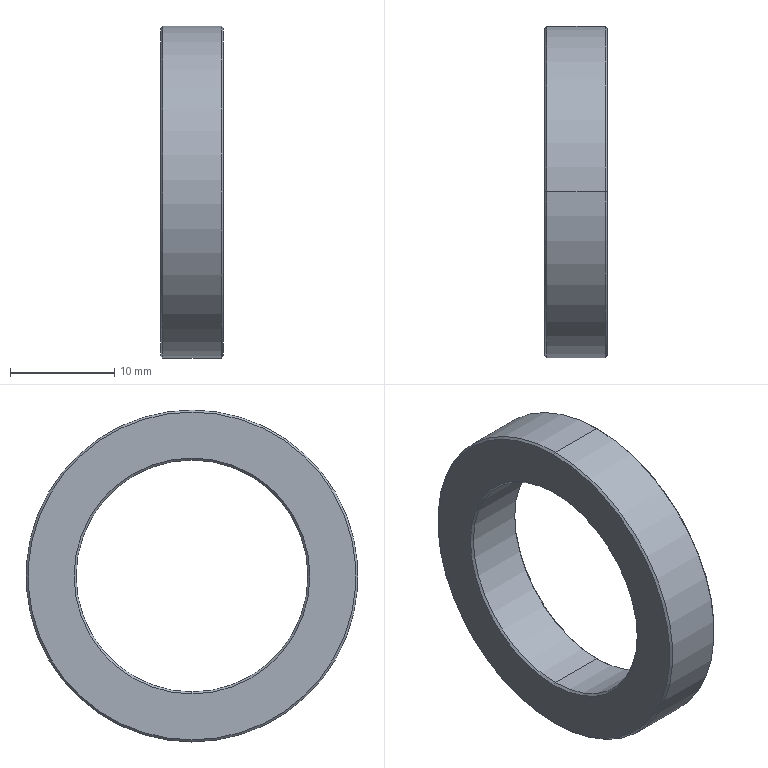Component | SolidWorks | XXXXX08-01-040514RotaryDriveShaft-1_XXXXX08-01-040515-1 | 1 solid | 14 faces | box 6 x 31.8 x 31.8 mm | volume 2436 mm3 | cone 8 | cylinder 4 | plane 2 | commonest cylinder face diameters 22.2 x2 31.8 x2 | material 45
build123d program:
from build123d import *

# Parameters (mm, degrees)
SKETCH1_R           = 15.9
SKETCH1_R_2         = 11.1
BOSS_EXTRUDE1_DEPTH = 3
CHAMFER1_SIZE       = 0.2


with BuildPart() as part:
    # Sketch1 → Boss-Extrude1 (new, symmetric)
    with BuildSketch(Plane(origin=(0, 0, 0), x_dir=(0, 0, -1), z_dir=(1, 0, 0))):
        Circle(SKETCH1_R)
        Circle(SKETCH1_R_2, mode=Mode.SUBTRACT)
    extrude(amount=BOSS_EXTRUDE1_DEPTH, both=True)

    # Chamfer1
    chamfer1_edges = [part.edges().sort_by_distance(p)[0] for p in [
        (-3, 0, 15.9),
        (3, 0, 15.9),
        (-3, 0, 11.1),
        (3, 0, 11.1),
    ]]
    chamfer(chamfer1_edges, length=CHAMFER1_SIZE)


solid = part.part

# Placed as in the assembly
solid = solid.moved(Location((-32.7, 0, 0), (0, 0, 0)))
STEP:
#1=COLOUR_RGB('',0.7922,0.8196,0.9333);
#2=FILL_AREA_STYLE_COLOUR('',#1);
#3=FILL_AREA_STYLE('',(#2));
#4=SURFACE_STYLE_FILL_AREA(#3);
#5=SURFACE_SIDE_STYLE('',(#4));
#6=SURFACE_STYLE_USAGE(.BOTH.,#5);
#7=PRESENTATION_STYLE_ASSIGNMENT((#6));
#8=CARTESIAN_POINT('',(-1.177,0.,0.437));
#9=VERTEX_POINT('',#8);
#10=CARTESIAN_POINT('',(-1.177,0.,-0.437));
#11=VERTEX_POINT('',#10);
#12=CARTESIAN_POINT('',(-1.177,0.,-0.));
#13=DIRECTION('',(1.,0.,0.));
#14=DIRECTION('',(0.,0.,-1.));
#15=AXIS2_PLACEMENT_3D('',#12,#13,#14);
#16=CIRCLE('',#15,0.437);
#17=EDGE_CURVE('',#9,#11,#16,.T.);
#18=ORIENTED_EDGE('',*,*,#17,.F.);
#19=CARTESIAN_POINT('',(-1.169,0.,0.4449));
#20=VERTEX_POINT('',#19);
#21=CARTESIAN_POINT('',(-1.177,0.,0.437));
#22=DIRECTION('',(0.7071,0.,0.7071));
#23=VECTOR('',#22,39.37);
#24=LINE('',#21,#23);
#25=EDGE_CURVE('',#9,#20,#24,.T.);
#26=ORIENTED_EDGE('',*,*,#25,.T.);
#27=CARTESIAN_POINT('',(-1.169,0.,-0.4449));
#28=VERTEX_POINT('',#27);
#29=CARTESIAN_POINT('',(-1.169,0.,-0.));
#30=DIRECTION('',(-1.,0.,0.));
#31=DIRECTION('',(0.,0.,-1.));
#32=AXIS2_PLACEMENT_3D('',#29,#30,#31);
#33=CIRCLE('',#32,0.4449);
#34=EDGE_CURVE('',#28,#20,#33,.T.);
#35=ORIENTED_EDGE('',*,*,#34,.F.);
#36=CARTESIAN_POINT('',(-1.177,0.,-0.437));
#37=DIRECTION('',(0.7071,0.,-0.7071));
#38=VECTOR('',#37,39.37);
#39=LINE('',#36,#38);
#40=EDGE_CURVE('',#11,#28,#39,.T.);
#41=ORIENTED_EDGE('',*,*,#40,.F.);
#42=EDGE_LOOP('',(#18,#26,#35,#41));
#43=FACE_OUTER_BOUND('',#42,.T.);
#44=CARTESIAN_POINT('',(-1.177,0.,-0.));
#45=DIRECTION('',(1.,0.,0.));
#46=DIRECTION('',(0.,0.,-1.));
#47=AXIS2_PLACEMENT_3D('',#44,#45,#46);
#48=CONICAL_SURFACE('',#47,0.437,0.7854);
#49=ADVANCED_FACE('',(#43),#48,.F.);
#50=CARTESIAN_POINT('',(-1.398,0.,-0.437));
#51=VERTEX_POINT('',#50);
#52=CARTESIAN_POINT('',(-1.398,0.,0.437));
#53=VERTEX_POINT('',#52);
#54=CARTESIAN_POINT('',(-1.398,0.,-0.));
#55=DIRECTION('',(-1.,0.,0.));
#56=DIRECTION('',(0.,0.,-1.));
#57=AXIS2_PLACEMENT_3D('',#54,#55,#56);
#58=CIRCLE('',#57,0.437);
#59=EDGE_CURVE('',#51,#53,#58,.T.);
#60=ORIENTED_EDGE('',*,*,#59,.F.);
#61=CARTESIAN_POINT('',(-1.406,0.,-0.4449));
#62=VERTEX_POINT('',#61);
#63=CARTESIAN_POINT('',(-1.406,0.,-0.4449));
#64=DIRECTION('',(-0.7071,0.,-0.7071));
#65=VECTOR('',#64,39.37);
#66=LINE('',#63,#65);
#67=EDGE_CURVE('',#51,#62,#66,.T.);
#68=ORIENTED_EDGE('',*,*,#67,.T.);
#69=CARTESIAN_POINT('',(-1.406,0.,0.4449));
#70=VERTEX_POINT('',#69);
#71=CARTESIAN_POINT('',(-1.406,0.,-0.));
#72=DIRECTION('',(1.,0.,0.));
#73=DIRECTION('',(0.,0.,-1.));
#74=AXIS2_PLACEMENT_3D('',#71,#72,#73);
#75=CIRCLE('',#74,0.4449);
#76=EDGE_CURVE('',#70,#62,#75,.T.);
#77=ORIENTED_EDGE('',*,*,#76,.F.);
#78=CARTESIAN_POINT('',(-1.406,0.,0.4449));
#79=DIRECTION('',(-0.7071,0.,0.7071));
#80=VECTOR('',#79,39.37);
#81=LINE('',#78,#80);
#82=EDGE_CURVE('',#53,#70,#81,.T.);
#83=ORIENTED_EDGE('',*,*,#82,.F.);
#84=EDGE_LOOP('',(#60,#68,#77,#83));
#85=FACE_OUTER_BOUND('',#84,.T.);
#86=CARTESIAN_POINT('',(-1.406,0.,-0.));
#87=DIRECTION('',(-1.,0.,0.));
#88=DIRECTION('',(0.,0.,1.));
#89=AXIS2_PLACEMENT_3D('',#86,#87,#88);
#90=CONICAL_SURFACE('',#89,0.4449,0.7854);
#91=ADVANCED_FACE('',(#85),#90,.F.);
#92=CARTESIAN_POINT('',(-1.169,0.,-0.6181));
#93=VERTEX_POINT('',#92);
#94=CARTESIAN_POINT('',(-1.169,0.,0.6181));
#95=VERTEX_POINT('',#94);
#96=CARTESIAN_POINT('',(-1.169,0.,-0.));
#97=DIRECTION('',(1.,0.,0.));
#98=DIRECTION('',(0.,0.,-1.));
#99=AXIS2_PLACEMENT_3D('',#96,#97,#98);
#100=CIRCLE('',#99,0.6181);
#101=EDGE_CURVE('',#93,#95,#100,.T.);
#102=ORIENTED_EDGE('',*,*,#101,.F.);
#103=CARTESIAN_POINT('',(-1.177,0.,-0.626));
#104=VERTEX_POINT('',#103);
#105=CARTESIAN_POINT('',(-1.169,0.,-0.6181));
#106=DIRECTION('',(-0.7071,0.,-0.7071));
#107=VECTOR('',#106,39.37);
#108=LINE('',#105,#107);
#109=EDGE_CURVE('',#93,#104,#108,.T.);
#110=ORIENTED_EDGE('',*,*,#109,.T.);
#111=CARTESIAN_POINT('',(-1.177,0.,0.626));
#112=VERTEX_POINT('',#111);
#113=CARTESIAN_POINT('',(-1.177,0.,-0.));
#114=DIRECTION('',(-1.,0.,0.));
#115=DIRECTION('',(0.,0.,-1.));
#116=AXIS2_PLACEMENT_3D('',#113,#114,#115);
#117=CIRCLE('',#116,0.626);
#118=EDGE_CURVE('',#112,#104,#117,.T.);
#119=ORIENTED_EDGE('',*,*,#118,.F.);
#120=CARTESIAN_POINT('',(-1.169,0.,0.6181));
#121=DIRECTION('',(-0.7071,0.,0.7071));
#122=VECTOR('',#121,39.37);
#123=LINE('',#120,#122);
#124=EDGE_CURVE('',#95,#112,#123,.T.);
#125=ORIENTED_EDGE('',*,*,#124,.F.);
#126=EDGE_LOOP('',(#102,#110,#119,#125));
#127=FACE_OUTER_BOUND('',#126,.T.);
#128=CARTESIAN_POINT('',(-1.169,0.,-0.));
#129=DIRECTION('',(-1.,0.,0.));
#130=DIRECTION('',(0.,0.,1.));
#131=AXIS2_PLACEMENT_3D('',#128,#129,#130);
#132=CONICAL_SURFACE('',#131,0.6181,0.7854);
#133=ADVANCED_FACE('',(#127),#132,.T.);
#134=CARTESIAN_POINT('',(-1.406,0.,0.6181));
#135=VERTEX_POINT('',#134);
#136=CARTESIAN_POINT('',(-1.406,0.,-0.6181));
#137=VERTEX_POINT('',#136);
#138=CARTESIAN_POINT('',(-1.406,0.,-0.));
#139=DIRECTION('',(-1.,0.,0.));
#140=DIRECTION('',(0.,0.,-1.));
#141=AXIS2_PLACEMENT_3D('',#138,#139,#140);
#142=CIRCLE('',#141,0.6181);
#143=EDGE_CURVE('',#135,#137,#142,.T.);
#144=ORIENTED_EDGE('',*,*,#143,.F.);
#145=CARTESIAN_POINT('',(-1.398,0.,0.626));
#146=VERTEX_POINT('',#145);
#147=CARTESIAN_POINT('',(-1.398,0.,0.626));
#148=DIRECTION('',(0.7071,0.,0.7071));
#149=VECTOR('',#148,39.37);
#150=LINE('',#147,#149);
#151=EDGE_CURVE('',#135,#146,#150,.T.);
#152=ORIENTED_EDGE('',*,*,#151,.T.);
#153=CARTESIAN_POINT('',(-1.398,0.,-0.626));
#154=VERTEX_POINT('',#153);
#155=CARTESIAN_POINT('',(-1.398,0.,-0.));
#156=DIRECTION('',(1.,0.,0.));
#157=DIRECTION('',(0.,0.,-1.));
#158=AXIS2_PLACEMENT_3D('',#155,#156,#157);
#159=CIRCLE('',#158,0.626);
#160=EDGE_CURVE('',#154,#146,#159,.T.);
#161=ORIENTED_EDGE('',*,*,#160,.F.);
#162=CARTESIAN_POINT('',(-1.398,0.,-0.626));
#163=DIRECTION('',(0.7071,0.,-0.7071));
#164=VECTOR('',#163,39.37);
#165=LINE('',#162,#164);
#166=EDGE_CURVE('',#137,#154,#165,.T.);
#167=ORIENTED_EDGE('',*,*,#166,.F.);
#168=EDGE_LOOP('',(#144,#152,#161,#167));
#169=FACE_OUTER_BOUND('',#168,.T.);
#170=CARTESIAN_POINT('',(-1.398,0.,-0.));
#171=DIRECTION('',(1.,0.,0.));
#172=DIRECTION('',(0.,0.,-1.));
#173=AXIS2_PLACEMENT_3D('',#170,#171,#172);
#174=CONICAL_SURFACE('',#173,0.626,0.7854);
#175=ADVANCED_FACE('',(#169),#174,.T.);
#176=ORIENTED_EDGE('',*,*,#17,.T.);
#177=CARTESIAN_POINT('',(-1.169,0.,-0.437));
#178=DIRECTION('',(-1.,0.,0.));
#179=VECTOR('',#178,39.37);
#180=LINE('',#177,#179);
#181=EDGE_CURVE('',#11,#51,#180,.T.);
#182=ORIENTED_EDGE('',*,*,#181,.T.);
#183=ORIENTED_EDGE('',*,*,#59,.T.);
#184=CARTESIAN_POINT('',(-1.169,0.,0.437));
#185=DIRECTION('',(-1.,0.,0.));
#186=VECTOR('',#185,39.37);
#187=LINE('',#184,#186);
#188=EDGE_CURVE('',#9,#53,#187,.T.);
#189=ORIENTED_EDGE('',*,*,#188,.F.);
#190=EDGE_LOOP('',(#176,#182,#183,#189));
#191=FACE_OUTER_BOUND('',#190,.T.);
#192=CARTESIAN_POINT('',(-1.169,0.,-0.));
#193=DIRECTION('',(-1.,0.,0.));
#194=DIRECTION('',(0.,0.,1.));
#195=AXIS2_PLACEMENT_3D('',#192,#193,#194);
#196=CYLINDRICAL_SURFACE('',#195,0.437);
#197=ADVANCED_FACE('',(#191),#196,.F.);
#198=ORIENTED_EDGE('',*,*,#118,.T.);
#199=CARTESIAN_POINT('',(-1.169,0.,-0.626));
#200=DIRECTION('',(-1.,0.,0.));
#201=VECTOR('',#200,39.37);
#202=LINE('',#199,#201);
#203=EDGE_CURVE('',#104,#154,#202,.T.);
#204=ORIENTED_EDGE('',*,*,#203,.T.);
#205=ORIENTED_EDGE('',*,*,#160,.T.);
#206=CARTESIAN_POINT('',(-1.169,0.,0.626));
#207=DIRECTION('',(-1.,0.,0.));
#208=VECTOR('',#207,39.37);
#209=LINE('',#206,#208);
#210=EDGE_CURVE('',#112,#146,#209,.T.);
#211=ORIENTED_EDGE('',*,*,#210,.F.);
#212=EDGE_LOOP('',(#198,#204,#205,#211));
#213=FACE_OUTER_BOUND('',#212,.T.);
#214=CARTESIAN_POINT('',(-1.169,0.,-0.));
#215=DIRECTION('',(-1.,0.,0.));
#216=DIRECTION('',(0.,0.,1.));
#217=AXIS2_PLACEMENT_3D('',#214,#215,#216);
#218=CYLINDRICAL_SURFACE('',#217,0.626);
#219=ADVANCED_FACE('',(#213),#218,.T.);
#220=CARTESIAN_POINT('',(-1.169,0.,-0.));
#221=DIRECTION('',(1.,0.,0.));
#222=DIRECTION('',(0.,0.,-1.));
#223=AXIS2_PLACEMENT_3D('',#220,#221,#222);
#224=CIRCLE('',#223,0.6181);
#225=EDGE_CURVE('',#95,#93,#224,.T.);
#226=ORIENTED_EDGE('',*,*,#225,.T.);
#227=ORIENTED_EDGE('',*,*,#101,.T.);
#228=EDGE_LOOP('',(#226,#227));
#229=FACE_OUTER_BOUND('',#228,.T.);
#230=ORIENTED_EDGE('',*,*,#34,.T.);
#231=CARTESIAN_POINT('',(-1.169,0.,-0.));
#232=DIRECTION('',(-1.,0.,0.));
#233=DIRECTION('',(0.,0.,-1.));
#234=AXIS2_PLACEMENT_3D('',#231,#232,#233);
#235=CIRCLE('',#234,0.4449);
#236=EDGE_CURVE('',#20,#28,#235,.T.);
#237=ORIENTED_EDGE('',*,*,#236,.T.);
#238=EDGE_LOOP('',(#230,#237));
#239=FACE_BOUND('',#238,.T.);
#240=CARTESIAN_POINT('',(-1.169,0.,-0.));
#241=DIRECTION('',(1.,0.,0.));
#242=DIRECTION('',(0.,0.,-1.));
#243=AXIS2_PLACEMENT_3D('',#240,#241,#242);
#244=PLANE('',#243);
#245=ADVANCED_FACE('',(#229,#239),#244,.T.);
#246=CARTESIAN_POINT('',(-1.406,0.,-0.));
#247=DIRECTION('',(-1.,0.,0.));
#248=DIRECTION('',(0.,0.,-1.));
#249=AXIS2_PLACEMENT_3D('',#246,#247,#248);
#250=CIRCLE('',#249,0.6181);
#251=EDGE_CURVE('',#137,#135,#250,.T.);
#252=ORIENTED_EDGE('',*,*,#251,.T.);
#253=ORIENTED_EDGE('',*,*,#143,.T.);
#254=EDGE_LOOP('',(#252,#253));
#255=FACE_OUTER_BOUND('',#254,.T.);
#256=ORIENTED_EDGE('',*,*,#76,.T.);
#257=CARTESIAN_POINT('',(-1.406,0.,-0.));
#258=DIRECTION('',(1.,0.,0.));
#259=DIRECTION('',(0.,0.,-1.));
#260=AXIS2_PLACEMENT_3D('',#257,#258,#259);
#261=CIRCLE('',#260,0.4449);
#262=EDGE_CURVE('',#62,#70,#261,.T.);
#263=ORIENTED_EDGE('',*,*,#262,.T.);
#264=EDGE_LOOP('',(#256,#263));
#265=FACE_BOUND('',#264,.T.);
#266=CARTESIAN_POINT('',(-1.406,0.,-0.));
#267=DIRECTION('',(1.,0.,0.));
#268=DIRECTION('',(0.,0.,-1.));
#269=AXIS2_PLACEMENT_3D('',#266,#267,#268);
#270=PLANE('',#269);
#271=ADVANCED_FACE('',(#255,#265),#270,.F.);
#272=ORIENTED_EDGE('',*,*,#203,.F.);
#273=CARTESIAN_POINT('',(-1.177,0.,-0.));
#274=DIRECTION('',(-1.,0.,0.));
#275=DIRECTION('',(0.,0.,-1.));
#276=AXIS2_PLACEMENT_3D('',#273,#274,#275);
#277=CIRCLE('',#276,0.626);
#278=EDGE_CURVE('',#104,#112,#277,.T.);
#279=ORIENTED_EDGE('',*,*,#278,.T.);
#280=ORIENTED_EDGE('',*,*,#210,.T.);
#281=CARTESIAN_POINT('',(-1.398,0.,-0.));
#282=DIRECTION('',(1.,0.,0.));
#283=DIRECTION('',(0.,0.,-1.));
#284=AXIS2_PLACEMENT_3D('',#281,#282,#283);
#285=CIRCLE('',#284,0.626);
#286=EDGE_CURVE('',#146,#154,#285,.T.);
#287=ORIENTED_EDGE('',*,*,#286,.T.);
#288=EDGE_LOOP('',(#272,#279,#280,#287));
#289=FACE_OUTER_BOUND('',#288,.T.);
#290=CARTESIAN_POINT('',(-1.169,0.,-0.));
#291=DIRECTION('',(-1.,0.,0.));
#292=DIRECTION('',(0.,0.,1.));
#293=AXIS2_PLACEMENT_3D('',#290,#291,#292);
#294=CYLINDRICAL_SURFACE('',#293,0.626);
#295=ADVANCED_FACE('',(#289),#294,.T.);
#296=ORIENTED_EDGE('',*,*,#181,.F.);
#297=CARTESIAN_POINT('',(-1.177,0.,-0.));
#298=DIRECTION('',(1.,0.,0.));
#299=DIRECTION('',(0.,0.,-1.));
#300=AXIS2_PLACEMENT_3D('',#297,#298,#299);
#301=CIRCLE('',#300,0.437);
#302=EDGE_CURVE('',#11,#9,#301,.T.);
#303=ORIENTED_EDGE('',*,*,#302,.T.);
#304=ORIENTED_EDGE('',*,*,#188,.T.);
#305=CARTESIAN_POINT('',(-1.398,0.,-0.));
#306=DIRECTION('',(-1.,0.,0.));
#307=DIRECTION('',(0.,0.,-1.));
#308=AXIS2_PLACEMENT_3D('',#305,#306,#307);
#309=CIRCLE('',#308,0.437);
#310=EDGE_CURVE('',#53,#51,#309,.T.);
#311=ORIENTED_EDGE('',*,*,#310,.T.);
#312=EDGE_LOOP('',(#296,#303,#304,#311));
#313=FACE_OUTER_BOUND('',#312,.T.);
#314=CARTESIAN_POINT('',(-1.169,0.,-0.));
#315=DIRECTION('',(-1.,0.,0.));
#316=DIRECTION('',(0.,0.,1.));
#317=AXIS2_PLACEMENT_3D('',#314,#315,#316);
#318=CYLINDRICAL_SURFACE('',#317,0.437);
#319=ADVANCED_FACE('',(#313),#318,.F.);
#320=ORIENTED_EDGE('',*,*,#151,.F.);
#321=ORIENTED_EDGE('',*,*,#251,.F.);
#322=ORIENTED_EDGE('',*,*,#166,.T.);
#323=ORIENTED_EDGE('',*,*,#286,.F.);
#324=EDGE_LOOP('',(#320,#321,#322,#323));
#325=FACE_OUTER_BOUND('',#324,.T.);
#326=CARTESIAN_POINT('',(-1.398,0.,-0.));
#327=DIRECTION('',(1.,0.,0.));
#328=DIRECTION('',(0.,0.,-1.));
#329=AXIS2_PLACEMENT_3D('',#326,#327,#328);
#330=CONICAL_SURFACE('',#329,0.626,0.7854);
#331=ADVANCED_FACE('',(#325),#330,.T.);
#332=ORIENTED_EDGE('',*,*,#109,.F.);
#333=ORIENTED_EDGE('',*,*,#225,.F.);
#334=ORIENTED_EDGE('',*,*,#124,.T.);
#335=ORIENTED_EDGE('',*,*,#278,.F.);
#336=EDGE_LOOP('',(#332,#333,#334,#335));
#337=FACE_OUTER_BOUND('',#336,.T.);
#338=CARTESIAN_POINT('',(-1.169,0.,-0.));
#339=DIRECTION('',(-1.,0.,0.));
#340=DIRECTION('',(0.,0.,1.));
#341=AXIS2_PLACEMENT_3D('',#338,#339,#340);
#342=CONICAL_SURFACE('',#341,0.6181,0.7854);
#343=ADVANCED_FACE('',(#337),#342,.T.);
#344=ORIENTED_EDGE('',*,*,#67,.F.);
#345=ORIENTED_EDGE('',*,*,#310,.F.);
#346=ORIENTED_EDGE('',*,*,#82,.T.);
#347=ORIENTED_EDGE('',*,*,#262,.F.);
#348=EDGE_LOOP('',(#344,#345,#346,#347));
#349=FACE_OUTER_BOUND('',#348,.T.);
#350=CARTESIAN_POINT('',(-1.406,0.,-0.));
#351=DIRECTION('',(-1.,0.,0.));
#352=DIRECTION('',(0.,0.,1.));
#353=AXIS2_PLACEMENT_3D('',#350,#351,#352);
#354=CONICAL_SURFACE('',#353,0.4449,0.7854);
#355=ADVANCED_FACE('',(#349),#354,.F.);
#356=ORIENTED_EDGE('',*,*,#25,.F.);
#357=ORIENTED_EDGE('',*,*,#302,.F.);
#358=ORIENTED_EDGE('',*,*,#40,.T.);
#359=ORIENTED_EDGE('',*,*,#236,.F.);
#360=EDGE_LOOP('',(#356,#357,#358,#359));
#361=FACE_OUTER_BOUND('',#360,.T.);
#362=CARTESIAN_POINT('',(-1.177,0.,-0.));
#363=DIRECTION('',(1.,0.,0.));
#364=DIRECTION('',(0.,0.,-1.));
#365=AXIS2_PLACEMENT_3D('',#362,#363,#364);
#366=CONICAL_SURFACE('',#365,0.437,0.7854);
#367=ADVANCED_FACE('',(#361),#366,.F.);
#368=CLOSED_SHELL('',(#49,#91,#133,#175,#197,#219,#245,#271,#295,#319,#331,#343,#355,#367));
#369=MANIFOLD_SOLID_BREP('',#368);
#370=STYLED_ITEM('',(#7),#369);
#371=PRESENTATION_LAYER_ASSIGNMENT('','',(#370));
#372=CARTESIAN_POINT('',(0.,0.,0.));
#373=DIRECTION('',(0.,0.,1.));
#374=DIRECTION('',(1.,0.,0.));
#375=AXIS2_PLACEMENT_3D('',#372,#373,#374);
#376=(LENGTH_UNIT()NAMED_UNIT(*)SI_UNIT($,.METRE.));
#377=LENGTH_MEASURE_WITH_UNIT(LENGTH_MEASURE(0.0254),#376);
#378=DIMENSIONAL_EXPONENTS(1.,0.,0.,0.,0.,0.,0.);
#379=(CONVERSION_BASED_UNIT('',#377)LENGTH_UNIT()NAMED_UNIT(#378));
#380=UNCERTAINTY_MEASURE_WITH_UNIT(LENGTH_MEASURE(0.00001),#379,'','');
#381=(NAMED_UNIT(*)PLANE_ANGLE_UNIT()SI_UNIT($,.RADIAN.));
#382=(NAMED_UNIT(*)SI_UNIT($,.STERADIAN.)SOLID_ANGLE_UNIT());
#383=(GEOMETRIC_REPRESENTATION_CONTEXT(3)GLOBAL_UNCERTAINTY_ASSIGNED_CONTEXT((#380))GLOBAL_UNIT_ASSIGNED_CONTEXT((#379,#381,#382))REPRESENTATION_CONTEXT('',''));
#384=ADVANCED_BREP_SHAPE_REPRESENTATION('',(#369,#375),#383);
#385=(LENGTH_UNIT()NAMED_UNIT(*)SI_UNIT($,.METRE.));
#386=LENGTH_MEASURE_WITH_UNIT(LENGTH_MEASURE(0.0254),#385);
#387=DIMENSIONAL_EXPONENTS(1.,0.,0.,0.,0.,0.,0.);
#388=(CONVERSION_BASED_UNIT('',#386)LENGTH_UNIT()NAMED_UNIT(#387));
#389=UNCERTAINTY_MEASURE_WITH_UNIT(LENGTH_MEASURE(0.00001),#388,'','');
#390=(NAMED_UNIT(*)PLANE_ANGLE_UNIT()SI_UNIT($,.RADIAN.));
#391=(NAMED_UNIT(*)SI_UNIT($,.STERADIAN.)SOLID_ANGLE_UNIT());
#392=(GEOMETRIC_REPRESENTATION_CONTEXT(3)GLOBAL_UNCERTAINTY_ASSIGNED_CONTEXT((#389))GLOBAL_UNIT_ASSIGNED_CONTEXT((#388,#390,#391))REPRESENTATION_CONTEXT('',''));
#393=MECHANICAL_DESIGN_GEOMETRIC_PRESENTATION_REPRESENTATION('',(#370),#392);